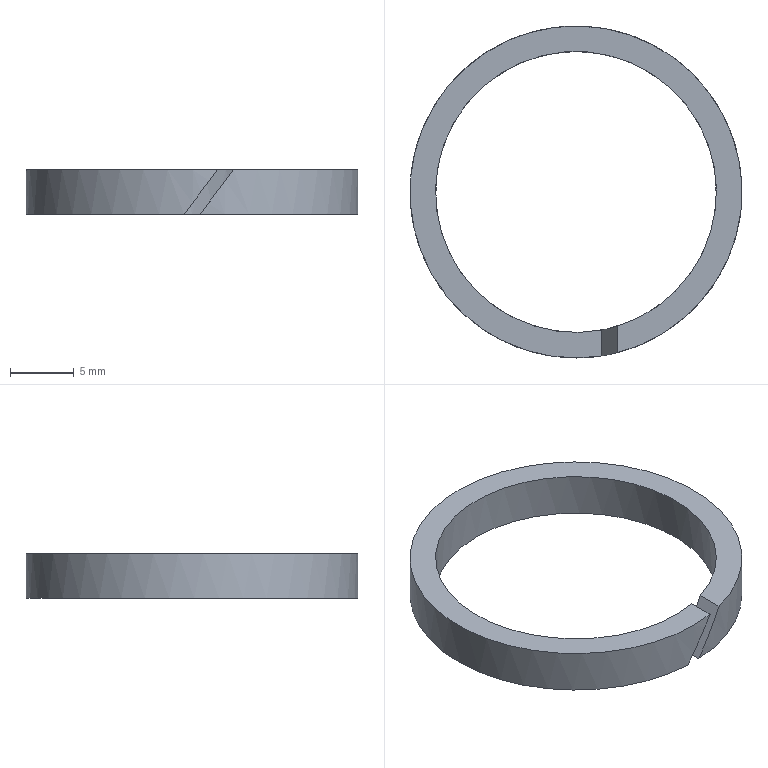Component | NX | PISTON_RING | 1 solid | 6 faces | volume 519 mm3 | plane 4 | cylinder 2 | commonest cylinder face diameters 26 x1 22 x1